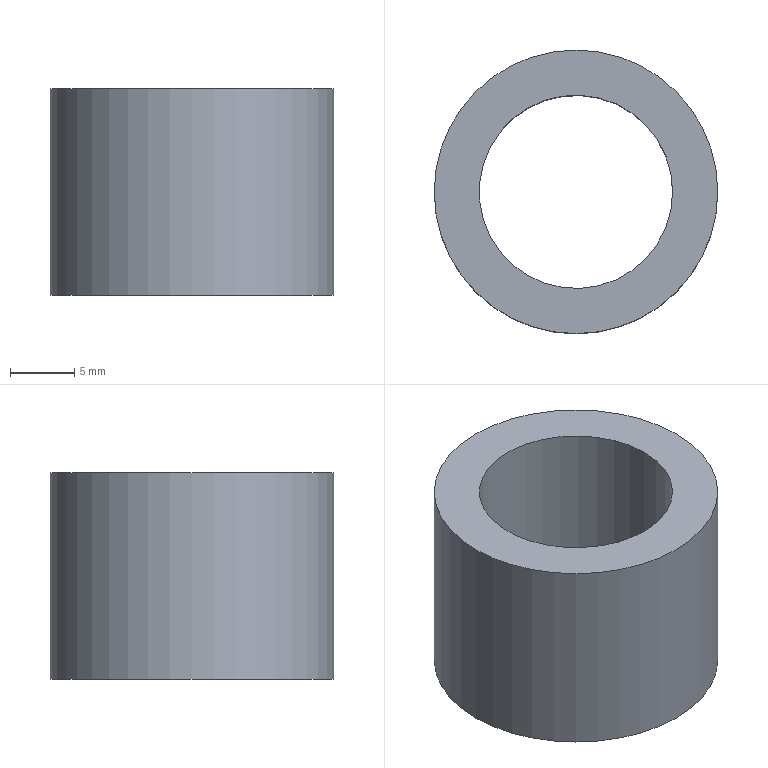Component | NX | BUSHING | 1 solid | 4 faces | box 22 x 22 x 16 mm | volume 3255 mm3 | cylinder 2 | plane 2 | commonest cylinder face diameters 22 x1 15 x1
STEP:
#1=CARTESIAN_POINT('',(0.,0.,0.));
#2=DIRECTION('',(0.,0.,1.));
#3=DIRECTION('',(1.,0.,0.));
#4=AXIS2_PLACEMENT_3D('',#1,#2,#3);
#5=CARTESIAN_POINT('',(11.,30.,-88.));
#6=VERTEX_POINT('',#5);
#7=CARTESIAN_POINT('',(-0.,30.,-88.));
#8=DIRECTION('',(0.,0.,1.));
#9=DIRECTION('',(1.,0.,0.));
#10=AXIS2_PLACEMENT_3D('',#7,#8,#9);
#11=CIRCLE('',#10,11.);
#12=CARTESIAN_POINT('',(-0.,30.,-88.));
#13=DIRECTION('',(0.,0.,-1.));
#14=DIRECTION('',(-1.,0.,0.));
#15=AXIS2_PLACEMENT_3D('',#12,#13,#14);
#16=CYLINDRICAL_SURFACE('',#15,11.);
#17=CARTESIAN_POINT('',(9.425,0.));
#18=DIRECTION('',(-1.,0.));
#19=VECTOR('',#18,1.);
#20=LINE('',#17,#19);
#21=(GEOMETRIC_REPRESENTATION_CONTEXT(2)PARAMETRIC_REPRESENTATION_CONTEXT()REPRESENTATION_CONTEXT('',''));
#22=DEFINITIONAL_REPRESENTATION('',(#20),#21);
#23=PCURVE('',#16,#22);
#24=CARTESIAN_POINT('',(-0.,30.,-88.));
#25=DIRECTION('',(0.,0.,1.));
#26=DIRECTION('',(1.,0.,0.));
#27=AXIS2_PLACEMENT_3D('',#24,#25,#26);
#28=PLANE('',#27);
#29=CARTESIAN_POINT('',(0.,0.));
#30=DIRECTION('',(1.,0.));
#31=AXIS2_PLACEMENT_2D('',#29,#30);
#32=CIRCLE('',#31,11.);
#33=(GEOMETRIC_REPRESENTATION_CONTEXT(2)PARAMETRIC_REPRESENTATION_CONTEXT()REPRESENTATION_CONTEXT('',''));
#34=DEFINITIONAL_REPRESENTATION('',(#32),#33);
#35=PCURVE('',#28,#34);
#36=SURFACE_CURVE('',#11,(#23,#35),.PCURVE_S1.);
#37=EDGE_CURVE('',#6,#6,#36,.T.);
#38=ORIENTED_EDGE('',*,*,#37,.F.);
#39=CARTESIAN_POINT('',(11.,30.,-104.));
#40=VERTEX_POINT('',#39);
#41=CARTESIAN_POINT('',(11.,30.,-88.));
#42=CARTESIAN_POINT('',(11.,30.,-104.));
#43=B_SPLINE_CURVE_WITH_KNOTS('',1,(#41,#42),.UNSPECIFIED.,.F.,.F.,(2,2),(0.,16.),.PIECEWISE_BEZIER_KNOTS.);
#44=CARTESIAN_POINT('',(9.425,0.));
#45=DIRECTION('',(0.,1.));
#46=VECTOR('',#45,1.);
#47=LINE('',#44,#46);
#48=(GEOMETRIC_REPRESENTATION_CONTEXT(2)PARAMETRIC_REPRESENTATION_CONTEXT()REPRESENTATION_CONTEXT('',''));
#49=DEFINITIONAL_REPRESENTATION('',(#47),#48);
#50=PCURVE('',#16,#49);
#51=CARTESIAN_POINT('',(3.142,0.));
#52=DIRECTION('',(0.,1.));
#53=VECTOR('',#52,1.);
#54=LINE('',#51,#53);
#55=(GEOMETRIC_REPRESENTATION_CONTEXT(2)PARAMETRIC_REPRESENTATION_CONTEXT()REPRESENTATION_CONTEXT('',''));
#56=DEFINITIONAL_REPRESENTATION('',(#54),#55);
#57=PCURVE('',#16,#56);
#58=SEAM_CURVE('',#43,(#50,#57),.PCURVE_S1.);
#59=EDGE_CURVE('',#6,#40,#58,.T.);
#60=ORIENTED_EDGE('',*,*,#59,.T.);
#61=CARTESIAN_POINT('',(-0.,30.,-104.));
#62=DIRECTION('',(0.,0.,1.));
#63=DIRECTION('',(1.,0.,0.));
#64=AXIS2_PLACEMENT_3D('',#61,#62,#63);
#65=CIRCLE('',#64,11.);
#66=CARTESIAN_POINT('',(9.425,16.));
#67=DIRECTION('',(-1.,0.));
#68=VECTOR('',#67,1.);
#69=LINE('',#66,#68);
#70=(GEOMETRIC_REPRESENTATION_CONTEXT(2)PARAMETRIC_REPRESENTATION_CONTEXT()REPRESENTATION_CONTEXT('',''));
#71=DEFINITIONAL_REPRESENTATION('',(#69),#70);
#72=PCURVE('',#16,#71);
#73=CARTESIAN_POINT('',(-0.,30.,-104.));
#74=DIRECTION('',(0.,0.,1.));
#75=DIRECTION('',(1.,0.,0.));
#76=AXIS2_PLACEMENT_3D('',#73,#74,#75);
#77=PLANE('',#76);
#78=CARTESIAN_POINT('',(0.,0.));
#79=DIRECTION('',(1.,0.));
#80=AXIS2_PLACEMENT_2D('',#78,#79);
#81=CIRCLE('',#80,11.);
#82=(GEOMETRIC_REPRESENTATION_CONTEXT(2)PARAMETRIC_REPRESENTATION_CONTEXT()REPRESENTATION_CONTEXT('',''));
#83=DEFINITIONAL_REPRESENTATION('',(#81),#82);
#84=PCURVE('',#77,#83);
#85=SURFACE_CURVE('',#65,(#72,#84),.PCURVE_S1.);
#86=EDGE_CURVE('',#40,#40,#85,.T.);
#87=ORIENTED_EDGE('',*,*,#86,.T.);
#88=ORIENTED_EDGE('',*,*,#59,.F.);
#89=EDGE_LOOP('',(#38,#60,#87,#88));
#90=FACE_BOUND('',#89,.T.);
#91=ADVANCED_FACE('',(#90),#16,.T.);
#92=CARTESIAN_POINT('',(7.5,30.,-88.));
#93=VERTEX_POINT('',#92);
#94=CARTESIAN_POINT('',(-0.,30.,-88.));
#95=DIRECTION('',(0.,0.,1.));
#96=DIRECTION('',(1.,0.,0.));
#97=AXIS2_PLACEMENT_3D('',#94,#95,#96);
#98=CIRCLE('',#97,7.5);
#99=CARTESIAN_POINT('',(-0.,30.,-88.));
#100=DIRECTION('',(0.,0.,-1.));
#101=DIRECTION('',(-1.,0.,0.));
#102=AXIS2_PLACEMENT_3D('',#99,#100,#101);
#103=CYLINDRICAL_SURFACE('',#102,7.5);
#104=CARTESIAN_POINT('',(9.425,0.));
#105=DIRECTION('',(-1.,0.));
#106=VECTOR('',#105,1.);
#107=LINE('',#104,#106);
#108=(GEOMETRIC_REPRESENTATION_CONTEXT(2)PARAMETRIC_REPRESENTATION_CONTEXT()REPRESENTATION_CONTEXT('',''));
#109=DEFINITIONAL_REPRESENTATION('',(#107),#108);
#110=PCURVE('',#103,#109);
#111=CARTESIAN_POINT('',(0.,0.));
#112=DIRECTION('',(1.,0.));
#113=AXIS2_PLACEMENT_2D('',#111,#112);
#114=CIRCLE('',#113,7.5);
#115=(GEOMETRIC_REPRESENTATION_CONTEXT(2)PARAMETRIC_REPRESENTATION_CONTEXT()REPRESENTATION_CONTEXT('',''));
#116=DEFINITIONAL_REPRESENTATION('',(#114),#115);
#117=PCURVE('',#28,#116);
#118=SURFACE_CURVE('',#98,(#110,#117),.PCURVE_S1.);
#119=EDGE_CURVE('',#93,#93,#118,.T.);
#120=ORIENTED_EDGE('',*,*,#119,.F.);
#121=CARTESIAN_POINT('',(7.5,30.,-104.));
#122=VERTEX_POINT('',#121);
#123=CARTESIAN_POINT('',(7.5,30.,-88.));
#124=CARTESIAN_POINT('',(7.5,30.,-104.));
#125=B_SPLINE_CURVE_WITH_KNOTS('',1,(#123,#124),.UNSPECIFIED.,.F.,.F.,(2,2),(0.,16.),.PIECEWISE_BEZIER_KNOTS.);
#126=CARTESIAN_POINT('',(9.425,0.));
#127=DIRECTION('',(0.,1.));
#128=VECTOR('',#127,1.);
#129=LINE('',#126,#128);
#130=(GEOMETRIC_REPRESENTATION_CONTEXT(2)PARAMETRIC_REPRESENTATION_CONTEXT()REPRESENTATION_CONTEXT('',''));
#131=DEFINITIONAL_REPRESENTATION('',(#129),#130);
#132=PCURVE('',#103,#131);
#133=CARTESIAN_POINT('',(3.142,0.));
#134=DIRECTION('',(0.,1.));
#135=VECTOR('',#134,1.);
#136=LINE('',#133,#135);
#137=(GEOMETRIC_REPRESENTATION_CONTEXT(2)PARAMETRIC_REPRESENTATION_CONTEXT()REPRESENTATION_CONTEXT('',''));
#138=DEFINITIONAL_REPRESENTATION('',(#136),#137);
#139=PCURVE('',#103,#138);
#140=SEAM_CURVE('',#125,(#132,#139),.PCURVE_S1.);
#141=EDGE_CURVE('',#93,#122,#140,.T.);
#142=ORIENTED_EDGE('',*,*,#141,.T.);
#143=CARTESIAN_POINT('',(-0.,30.,-104.));
#144=DIRECTION('',(0.,0.,1.));
#145=DIRECTION('',(1.,0.,0.));
#146=AXIS2_PLACEMENT_3D('',#143,#144,#145);
#147=CIRCLE('',#146,7.5);
#148=CARTESIAN_POINT('',(9.425,16.));
#149=DIRECTION('',(-1.,0.));
#150=VECTOR('',#149,1.);
#151=LINE('',#148,#150);
#152=(GEOMETRIC_REPRESENTATION_CONTEXT(2)PARAMETRIC_REPRESENTATION_CONTEXT()REPRESENTATION_CONTEXT('',''));
#153=DEFINITIONAL_REPRESENTATION('',(#151),#152);
#154=PCURVE('',#103,#153);
#155=CARTESIAN_POINT('',(0.,0.));
#156=DIRECTION('',(1.,0.));
#157=AXIS2_PLACEMENT_2D('',#155,#156);
#158=CIRCLE('',#157,7.5);
#159=(GEOMETRIC_REPRESENTATION_CONTEXT(2)PARAMETRIC_REPRESENTATION_CONTEXT()REPRESENTATION_CONTEXT('',''));
#160=DEFINITIONAL_REPRESENTATION('',(#158),#159);
#161=PCURVE('',#77,#160);
#162=SURFACE_CURVE('',#147,(#154,#161),.PCURVE_S1.);
#163=EDGE_CURVE('',#122,#122,#162,.T.);
#164=ORIENTED_EDGE('',*,*,#163,.T.);
#165=ORIENTED_EDGE('',*,*,#141,.F.);
#166=EDGE_LOOP('',(#120,#142,#164,#165));
#167=FACE_BOUND('',#166,.F.);
#168=ADVANCED_FACE('',(#167),#103,.F.);
#169=ORIENTED_EDGE('',*,*,#37,.T.);
#170=EDGE_LOOP('',(#169));
#171=FACE_BOUND('',#170,.T.);
#172=ORIENTED_EDGE('',*,*,#119,.F.);
#173=EDGE_LOOP('',(#172));
#174=FACE_BOUND('',#173,.T.);
#175=ADVANCED_FACE('',(#171,#174),#28,.T.);
#176=ORIENTED_EDGE('',*,*,#86,.F.);
#177=EDGE_LOOP('',(#176));
#178=FACE_BOUND('',#177,.T.);
#179=ORIENTED_EDGE('',*,*,#163,.T.);
#180=EDGE_LOOP('',(#179));
#181=FACE_BOUND('',#180,.T.);
#182=ADVANCED_FACE('',(#178,#181),#77,.F.);
#183=CLOSED_SHELL('',(#91,#168,#175,#182));
#184=MANIFOLD_SOLID_BREP('',#183);
#185=(LENGTH_UNIT()NAMED_UNIT(*)SI_UNIT(.MILLI.,.METRE.));
#186=UNCERTAINTY_MEASURE_WITH_UNIT(LENGTH_MEASURE(0.00001),#185,'','');
#187=(NAMED_UNIT(*)PLANE_ANGLE_UNIT()SI_UNIT($,.RADIAN.));
#188=(NAMED_UNIT(*)SI_UNIT($,.STERADIAN.)SOLID_ANGLE_UNIT());
#189=(GEOMETRIC_REPRESENTATION_CONTEXT(3)GLOBAL_UNCERTAINTY_ASSIGNED_CONTEXT((#186))GLOBAL_UNIT_ASSIGNED_CONTEXT((#185,#187,#188))REPRESENTATION_CONTEXT('',''));
#190=ADVANCED_BREP_SHAPE_REPRESENTATION('',(#4,#184),#189);